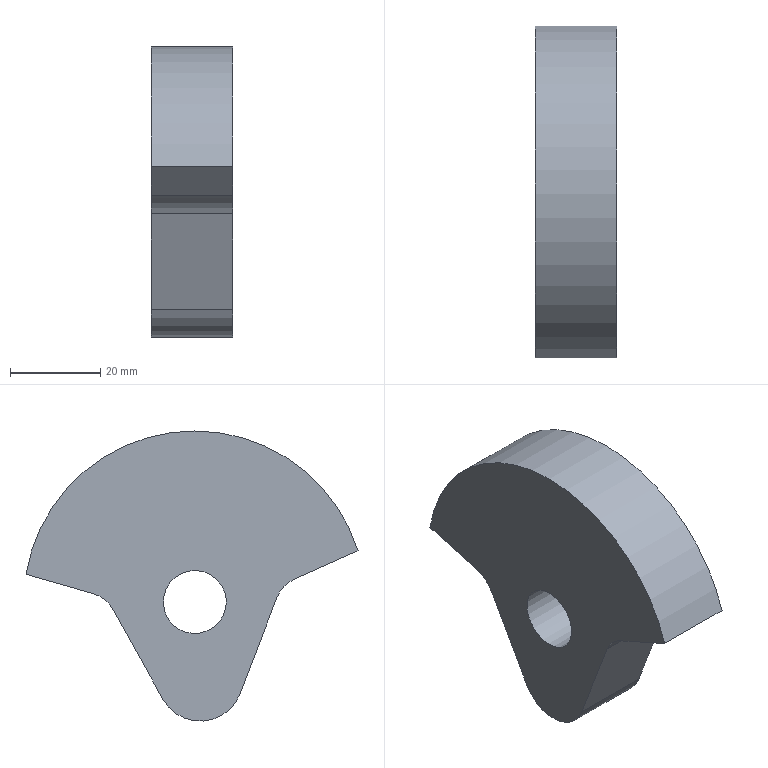Component | NX | TURNTABLE | 1 solid | 11 faces | box 18 x 73.75 x 64.46 mm | volume 45751 mm3 | plane 6 | cylinder 5 | commonest cylinder face diameters 14.905 x2 76 x1 19 x1 14 x1
STEP:
#1=CARTESIAN_POINT('',(0.,0.,0.));
#2=DIRECTION('',(0.,0.,1.));
#3=DIRECTION('',(1.,0.,0.));
#4=AXIS2_PLACEMENT_3D('',#1,#2,#3);
#5=CARTESIAN_POINT('',(-62.75,37.501,129.137));
#6=VERTEX_POINT('',#5);
#7=CARTESIAN_POINT('',(-62.75,-36.252,134.393));
#8=VERTEX_POINT('',#7);
#9=CARTESIAN_POINT('',(-62.75,0.,123.));
#10=DIRECTION('',(1.,0.,0.));
#11=DIRECTION('',(0.,0.9975,-0.07108));
#12=AXIS2_PLACEMENT_3D('',#9,#10,#11);
#13=CIRCLE('',#12,38.);
#14=CARTESIAN_POINT('',(-80.75,0.,123.));
#15=DIRECTION('',(1.,0.,0.));
#16=DIRECTION('',(0.,-0.07108,-0.9975));
#17=AXIS2_PLACEMENT_3D('',#14,#15,#16);
#18=CYLINDRICAL_SURFACE('',#17,38.);
#19=CARTESIAN_POINT('',(1.571,18.));
#20=DIRECTION('',(1.,0.));
#21=VECTOR('',#20,1.);
#22=LINE('',#19,#21);
#23=(GEOMETRIC_REPRESENTATION_CONTEXT(2)PARAMETRIC_REPRESENTATION_CONTEXT()REPRESENTATION_CONTEXT('',''));
#24=DEFINITIONAL_REPRESENTATION('',(#22),#23);
#25=PCURVE('',#18,#24);
#26=CARTESIAN_POINT('',(-62.75,0.,123.));
#27=DIRECTION('',(1.,0.,0.));
#28=DIRECTION('',(0.,-0.07108,-0.9975));
#29=AXIS2_PLACEMENT_3D('',#26,#27,#28);
#30=PLANE('',#29);
#31=CARTESIAN_POINT('',(0.,0.));
#32=DIRECTION('',(0.,1.));
#33=AXIS2_PLACEMENT_2D('',#31,#32);
#34=CIRCLE('',#33,38.);
#35=(GEOMETRIC_REPRESENTATION_CONTEXT(2)PARAMETRIC_REPRESENTATION_CONTEXT()REPRESENTATION_CONTEXT('',''));
#36=DEFINITIONAL_REPRESENTATION('',(#34),#35);
#37=PCURVE('',#30,#36);
#38=SURFACE_CURVE('',#13,(#25,#37),.PCURVE_S1.);
#39=EDGE_CURVE('',#6,#8,#38,.T.);
#40=ORIENTED_EDGE('',*,*,#39,.F.);
#41=CARTESIAN_POINT('',(-80.75,37.501,129.137));
#42=VERTEX_POINT('',#41);
#43=CARTESIAN_POINT('',(-80.75,37.501,129.137));
#44=DIRECTION('',(1.,0.,0.));
#45=VECTOR('',#44,1.);
#46=LINE('',#43,#45);
#47=CARTESIAN_POINT('',(1.804,0.));
#48=DIRECTION('',(0.,1.));
#49=VECTOR('',#48,1.);
#50=LINE('',#47,#49);
#51=(GEOMETRIC_REPRESENTATION_CONTEXT(2)PARAMETRIC_REPRESENTATION_CONTEXT()REPRESENTATION_CONTEXT('',''));
#52=DEFINITIONAL_REPRESENTATION('',(#50),#51);
#53=PCURVE('',#18,#52);
#54=CARTESIAN_POINT('',(-80.75,22.643,124.898));
#55=DIRECTION('',(0.,0.2744,-0.9616));
#56=DIRECTION('',(0.,-0.9616,-0.2744));
#57=AXIS2_PLACEMENT_3D('',#54,#55,#56);
#58=PLANE('',#57);
#59=CARTESIAN_POINT('',(-15.451,0.));
#60=DIRECTION('',(0.,-1.));
#61=VECTOR('',#60,1.);
#62=LINE('',#59,#61);
#63=(GEOMETRIC_REPRESENTATION_CONTEXT(2)PARAMETRIC_REPRESENTATION_CONTEXT()REPRESENTATION_CONTEXT('',''));
#64=DEFINITIONAL_REPRESENTATION('',(#62),#63);
#65=PCURVE('',#58,#64);
#66=SURFACE_CURVE('',#46,(#53,#65),.PCURVE_S1.);
#67=EDGE_CURVE('',#42,#6,#66,.T.);
#68=ORIENTED_EDGE('',*,*,#67,.F.);
#69=CARTESIAN_POINT('',(-80.75,-36.252,134.393));
#70=VERTEX_POINT('',#69);
#71=CARTESIAN_POINT('',(-80.75,0.,123.));
#72=DIRECTION('',(1.,0.,0.));
#73=DIRECTION('',(0.,0.9975,-0.07108));
#74=AXIS2_PLACEMENT_3D('',#71,#72,#73);
#75=CIRCLE('',#74,38.);
#76=CARTESIAN_POINT('',(1.571,0.));
#77=DIRECTION('',(1.,0.));
#78=VECTOR('',#77,1.);
#79=LINE('',#76,#78);
#80=(GEOMETRIC_REPRESENTATION_CONTEXT(2)PARAMETRIC_REPRESENTATION_CONTEXT()REPRESENTATION_CONTEXT('',''));
#81=DEFINITIONAL_REPRESENTATION('',(#79),#80);
#82=PCURVE('',#18,#81);
#83=CARTESIAN_POINT('',(-80.75,0.,123.));
#84=DIRECTION('',(1.,0.,0.));
#85=DIRECTION('',(0.,-0.07108,-0.9975));
#86=AXIS2_PLACEMENT_3D('',#83,#84,#85);
#87=PLANE('',#86);
#88=CARTESIAN_POINT('',(0.,0.));
#89=DIRECTION('',(0.,1.));
#90=AXIS2_PLACEMENT_2D('',#88,#89);
#91=CIRCLE('',#90,38.);
#92=(GEOMETRIC_REPRESENTATION_CONTEXT(2)PARAMETRIC_REPRESENTATION_CONTEXT()REPRESENTATION_CONTEXT('',''));
#93=DEFINITIONAL_REPRESENTATION('',(#91),#92);
#94=PCURVE('',#87,#93);
#95=SURFACE_CURVE('',#75,(#82,#94),.PCURVE_S1.);
#96=EDGE_CURVE('',#42,#70,#95,.T.);
#97=ORIENTED_EDGE('',*,*,#96,.T.);
#98=CARTESIAN_POINT('',(-80.75,-36.252,134.393));
#99=DIRECTION('',(1.,0.,0.));
#100=VECTOR('',#99,1.);
#101=LINE('',#98,#100);
#102=CARTESIAN_POINT('',(4.479,0.));
#103=DIRECTION('',(0.,1.));
#104=VECTOR('',#103,1.);
#105=LINE('',#102,#104);
#106=(GEOMETRIC_REPRESENTATION_CONTEXT(2)PARAMETRIC_REPRESENTATION_CONTEXT()REPRESENTATION_CONTEXT('',''));
#107=DEFINITIONAL_REPRESENTATION('',(#105),#106);
#108=PCURVE('',#18,#107);
#109=CARTESIAN_POINT('',(-80.75,-36.252,134.393));
#110=DIRECTION('',(0.,-0.4079,-0.913));
#111=DIRECTION('',(0.,-0.913,0.4079));
#112=AXIS2_PLACEMENT_3D('',#109,#110,#111);
#113=PLANE('',#112);
#114=CARTESIAN_POINT('',(0.,0.));
#115=DIRECTION('',(0.,-1.));
#116=VECTOR('',#115,1.);
#117=LINE('',#114,#116);
#118=(GEOMETRIC_REPRESENTATION_CONTEXT(2)PARAMETRIC_REPRESENTATION_CONTEXT()REPRESENTATION_CONTEXT('',''));
#119=DEFINITIONAL_REPRESENTATION('',(#117),#118);
#120=PCURVE('',#113,#119);
#121=SURFACE_CURVE('',#101,(#108,#120),.PCURVE_S1.);
#122=EDGE_CURVE('',#70,#8,#121,.T.);
#123=ORIENTED_EDGE('',*,*,#122,.T.);
#124=EDGE_LOOP('',(#40,#68,#97,#123));
#125=FACE_BOUND('',#124,.T.);
#126=ADVANCED_FACE('',(#125),#18,.T.);
#127=CARTESIAN_POINT('',(-62.75,-22.145,128.09));
#128=VERTEX_POINT('',#127);
#129=CARTESIAN_POINT('',(-62.75,-36.252,134.393));
#130=DIRECTION('',(0.,0.913,-0.4079));
#131=VECTOR('',#130,1.);
#132=LINE('',#129,#131);
#133=CARTESIAN_POINT('',(0.,-18.));
#134=DIRECTION('',(-1.,0.));
#135=VECTOR('',#134,1.);
#136=LINE('',#133,#135);
#137=(GEOMETRIC_REPRESENTATION_CONTEXT(2)PARAMETRIC_REPRESENTATION_CONTEXT()REPRESENTATION_CONTEXT('',''));
#138=DEFINITIONAL_REPRESENTATION('',(#136),#137);
#139=PCURVE('',#113,#138);
#140=CARTESIAN_POINT('',(-8.787,-36.97));
#141=DIRECTION('',(0.342,0.9397));
#142=VECTOR('',#141,1.);
#143=LINE('',#140,#142);
#144=(GEOMETRIC_REPRESENTATION_CONTEXT(2)PARAMETRIC_REPRESENTATION_CONTEXT()REPRESENTATION_CONTEXT('',''));
#145=DEFINITIONAL_REPRESENTATION('',(#143),#144);
#146=PCURVE('',#30,#145);
#147=SURFACE_CURVE('',#132,(#139,#146),.PCURVE_S1.);
#148=EDGE_CURVE('',#8,#128,#147,.T.);
#149=ORIENTED_EDGE('',*,*,#148,.F.);
#150=ORIENTED_EDGE('',*,*,#122,.F.);
#151=CARTESIAN_POINT('',(-80.75,-22.145,128.09));
#152=VERTEX_POINT('',#151);
#153=CARTESIAN_POINT('',(-80.75,-36.252,134.393));
#154=DIRECTION('',(0.,0.913,-0.4079));
#155=VECTOR('',#154,1.);
#156=LINE('',#153,#155);
#157=CARTESIAN_POINT('',(0.,0.));
#158=DIRECTION('',(-1.,0.));
#159=VECTOR('',#158,1.);
#160=LINE('',#157,#159);
#161=(GEOMETRIC_REPRESENTATION_CONTEXT(2)PARAMETRIC_REPRESENTATION_CONTEXT()REPRESENTATION_CONTEXT('',''));
#162=DEFINITIONAL_REPRESENTATION('',(#160),#161);
#163=PCURVE('',#113,#162);
#164=CARTESIAN_POINT('',(-8.787,-36.97));
#165=DIRECTION('',(0.342,0.9397));
#166=VECTOR('',#165,1.);
#167=LINE('',#164,#166);
#168=(GEOMETRIC_REPRESENTATION_CONTEXT(2)PARAMETRIC_REPRESENTATION_CONTEXT()REPRESENTATION_CONTEXT('',''));
#169=DEFINITIONAL_REPRESENTATION('',(#167),#168);
#170=PCURVE('',#87,#169);
#171=SURFACE_CURVE('',#156,(#163,#170),.PCURVE_S1.);
#172=EDGE_CURVE('',#70,#152,#171,.T.);
#173=ORIENTED_EDGE('',*,*,#172,.T.);
#174=CARTESIAN_POINT('',(-80.75,-22.145,128.09));
#175=DIRECTION('',(1.,0.,0.));
#176=VECTOR('',#175,1.);
#177=LINE('',#174,#176);
#178=CARTESIAN_POINT('',(-15.451,0.));
#179=DIRECTION('',(0.,-1.));
#180=VECTOR('',#179,1.);
#181=LINE('',#178,#180);
#182=(GEOMETRIC_REPRESENTATION_CONTEXT(2)PARAMETRIC_REPRESENTATION_CONTEXT()REPRESENTATION_CONTEXT('',''));
#183=DEFINITIONAL_REPRESENTATION('',(#181),#182);
#184=PCURVE('',#113,#183);
#185=CARTESIAN_POINT('',(-80.75,-25.186,121.286));
#186=DIRECTION('',(1.,0.,0.));
#187=DIRECTION('',(0.,-0.07108,-0.9975));
#188=AXIS2_PLACEMENT_3D('',#185,#186,#187);
#189=CYLINDRICAL_SURFACE('',#188,7.452);
#190=CARTESIAN_POINT('',(2.793,0.));
#191=DIRECTION('',(0.,1.));
#192=VECTOR('',#191,1.);
#193=LINE('',#190,#192);
#194=(GEOMETRIC_REPRESENTATION_CONTEXT(2)PARAMETRIC_REPRESENTATION_CONTEXT()REPRESENTATION_CONTEXT('',''));
#195=DEFINITIONAL_REPRESENTATION('',(#193),#194);
#196=PCURVE('',#189,#195);
#197=SURFACE_CURVE('',#177,(#184,#196),.PCURVE_S1.);
#198=EDGE_CURVE('',#152,#128,#197,.T.);
#199=ORIENTED_EDGE('',*,*,#198,.T.);
#200=EDGE_LOOP('',(#149,#150,#173,#199));
#201=FACE_BOUND('',#200,.T.);
#202=ADVANCED_FACE('',(#201),#113,.T.);
#203=CARTESIAN_POINT('',(-80.75,-18.225,123.947));
#204=VERTEX_POINT('',#203);
#205=CARTESIAN_POINT('',(-62.75,-18.225,123.947));
#206=VERTEX_POINT('',#205);
#207=CARTESIAN_POINT('',(-80.75,-18.225,123.947));
#208=DIRECTION('',(1.,0.,0.));
#209=VECTOR('',#208,1.);
#210=LINE('',#207,#209);
#211=CARTESIAN_POINT('',(2.007,0.));
#212=DIRECTION('',(0.,1.));
#213=VECTOR('',#212,1.);
#214=LINE('',#211,#213);
#215=(GEOMETRIC_REPRESENTATION_CONTEXT(2)PARAMETRIC_REPRESENTATION_CONTEXT()REPRESENTATION_CONTEXT('',''));
#216=DEFINITIONAL_REPRESENTATION('',(#214),#215);
#217=PCURVE('',#189,#216);
#218=CARTESIAN_POINT('',(-80.75,-18.225,123.947));
#219=DIRECTION('',(0.,-0.9341,-0.3571));
#220=DIRECTION('',(0.,-0.3571,0.9341));
#221=AXIS2_PLACEMENT_3D('',#218,#219,#220);
#222=PLANE('',#221);
#223=CARTESIAN_POINT('',(0.,0.));
#224=DIRECTION('',(0.,-1.));
#225=VECTOR('',#224,1.);
#226=LINE('',#223,#225);
#227=(GEOMETRIC_REPRESENTATION_CONTEXT(2)PARAMETRIC_REPRESENTATION_CONTEXT()REPRESENTATION_CONTEXT('',''));
#228=DEFINITIONAL_REPRESENTATION('',(#226),#227);
#229=PCURVE('',#222,#228);
#230=SURFACE_CURVE('',#210,(#217,#229),.PCURVE_S1.);
#231=EDGE_CURVE('',#204,#206,#230,.T.);
#232=ORIENTED_EDGE('',*,*,#231,.F.);
#233=CARTESIAN_POINT('',(-80.75,-25.186,121.286));
#234=DIRECTION('',(-1.,0.,0.));
#235=DIRECTION('',(0.,0.9975,-0.07108));
#236=AXIS2_PLACEMENT_3D('',#233,#234,#235);
#237=CIRCLE('',#236,7.452);
#238=CARTESIAN_POINT('',(7.854,0.));
#239=DIRECTION('',(-1.,0.));
#240=VECTOR('',#239,1.);
#241=LINE('',#238,#240);
#242=(GEOMETRIC_REPRESENTATION_CONTEXT(2)PARAMETRIC_REPRESENTATION_CONTEXT()REPRESENTATION_CONTEXT('',''));
#243=DEFINITIONAL_REPRESENTATION('',(#241),#242);
#244=PCURVE('',#189,#243);
#245=CARTESIAN_POINT('',(3.5,-17.548));
#246=CARTESIAN_POINT('',(16.408,-17.548));
#247=CARTESIAN_POINT('',(9.954,-28.726));
#248=CARTESIAN_POINT('',(3.5,-39.905));
#249=CARTESIAN_POINT('',(-2.954,-28.726));
#250=CARTESIAN_POINT('',(-9.408,-17.548));
#251=CARTESIAN_POINT('',(3.5,-17.548));
#252=(BOUNDED_CURVE()B_SPLINE_CURVE(2,(#245,#246,#247,#248,#249,#250,#251),.UNSPECIFIED.,.T.,.F.)B_SPLINE_CURVE_WITH_KNOTS((1,2,2,2,2,1),(-2.094,0.,2.094,4.189,6.283,8.378),.UNSPECIFIED.)CURVE()GEOMETRIC_REPRESENTATION_ITEM()RATIONAL_B_SPLINE_CURVE((1.,0.5,1.,0.5,1.,0.5,1.))REPRESENTATION_ITEM(''));
#253=(GEOMETRIC_REPRESENTATION_CONTEXT(2)PARAMETRIC_REPRESENTATION_CONTEXT()REPRESENTATION_CONTEXT('',''));
#254=DEFINITIONAL_REPRESENTATION('',(#252),#253);
#255=PCURVE('',#87,#254);
#256=SURFACE_CURVE('',#237,(#244,#255),.PCURVE_S1.);
#257=EDGE_CURVE('',#152,#204,#256,.T.);
#258=ORIENTED_EDGE('',*,*,#257,.F.);
#259=ORIENTED_EDGE('',*,*,#198,.T.);
#260=CARTESIAN_POINT('',(-62.75,-25.186,121.286));
#261=DIRECTION('',(-1.,0.,0.));
#262=DIRECTION('',(0.,0.9975,-0.07108));
#263=AXIS2_PLACEMENT_3D('',#260,#261,#262);
#264=CIRCLE('',#263,7.452);
#265=CARTESIAN_POINT('',(7.854,18.));
#266=DIRECTION('',(-1.,0.));
#267=VECTOR('',#266,1.);
#268=LINE('',#265,#267);
#269=(GEOMETRIC_REPRESENTATION_CONTEXT(2)PARAMETRIC_REPRESENTATION_CONTEXT()REPRESENTATION_CONTEXT('',''));
#270=DEFINITIONAL_REPRESENTATION('',(#268),#269);
#271=PCURVE('',#189,#270);
#272=CARTESIAN_POINT('',(3.5,-17.548));
#273=CARTESIAN_POINT('',(16.408,-17.548));
#274=CARTESIAN_POINT('',(9.954,-28.726));
#275=CARTESIAN_POINT('',(3.5,-39.905));
#276=CARTESIAN_POINT('',(-2.954,-28.726));
#277=CARTESIAN_POINT('',(-9.408,-17.548));
#278=CARTESIAN_POINT('',(3.5,-17.548));
#279=(BOUNDED_CURVE()B_SPLINE_CURVE(2,(#272,#273,#274,#275,#276,#277,#278),.UNSPECIFIED.,.T.,.F.)B_SPLINE_CURVE_WITH_KNOTS((1,2,2,2,2,1),(-2.094,0.,2.094,4.189,6.283,8.378),.UNSPECIFIED.)CURVE()GEOMETRIC_REPRESENTATION_ITEM()RATIONAL_B_SPLINE_CURVE((1.,0.5,1.,0.5,1.,0.5,1.))REPRESENTATION_ITEM(''));
#280=(GEOMETRIC_REPRESENTATION_CONTEXT(2)PARAMETRIC_REPRESENTATION_CONTEXT()REPRESENTATION_CONTEXT('',''));
#281=DEFINITIONAL_REPRESENTATION('',(#279),#280);
#282=PCURVE('',#30,#281);
#283=SURFACE_CURVE('',#264,(#271,#282),.PCURVE_S1.);
#284=EDGE_CURVE('',#128,#206,#283,.T.);
#285=ORIENTED_EDGE('',*,*,#284,.T.);
#286=EDGE_LOOP('',(#232,#258,#259,#285));
#287=FACE_BOUND('',#286,.F.);
#288=ADVANCED_FACE('',(#287),#189,.F.);
#289=CARTESIAN_POINT('',(-62.75,-10.082,102.65));
#290=VERTEX_POINT('',#289);
#291=CARTESIAN_POINT('',(-62.75,-18.225,123.947));
#292=DIRECTION('',(0.,0.3571,-0.9341));
#293=VECTOR('',#292,1.);
#294=LINE('',#291,#293);
#295=CARTESIAN_POINT('',(0.,-18.));
#296=DIRECTION('',(-1.,0.));
#297=VECTOR('',#296,1.);
#298=LINE('',#295,#297);
#299=(GEOMETRIC_REPRESENTATION_CONTEXT(2)PARAMETRIC_REPRESENTATION_CONTEXT()REPRESENTATION_CONTEXT('',''));
#300=DEFINITIONAL_REPRESENTATION('',(#298),#299);
#301=PCURVE('',#222,#300);
#302=CARTESIAN_POINT('',(0.3505,-18.246));
#303=DIRECTION('',(0.9063,0.4226));
#304=VECTOR('',#303,1.);
#305=LINE('',#302,#304);
#306=(GEOMETRIC_REPRESENTATION_CONTEXT(2)PARAMETRIC_REPRESENTATION_CONTEXT()REPRESENTATION_CONTEXT('',''));
#307=DEFINITIONAL_REPRESENTATION('',(#305),#306);
#308=PCURVE('',#30,#307);
#309=SURFACE_CURVE('',#294,(#301,#308),.PCURVE_S1.);
#310=EDGE_CURVE('',#206,#290,#309,.T.);
#311=ORIENTED_EDGE('',*,*,#310,.F.);
#312=ORIENTED_EDGE('',*,*,#231,.F.);
#313=CARTESIAN_POINT('',(-80.75,-10.082,102.65));
#314=VERTEX_POINT('',#313);
#315=CARTESIAN_POINT('',(-80.75,-18.225,123.947));
#316=DIRECTION('',(0.,0.3571,-0.9341));
#317=VECTOR('',#316,1.);
#318=LINE('',#315,#317);
#319=CARTESIAN_POINT('',(0.,0.));
#320=DIRECTION('',(-1.,0.));
#321=VECTOR('',#320,1.);
#322=LINE('',#319,#321);
#323=(GEOMETRIC_REPRESENTATION_CONTEXT(2)PARAMETRIC_REPRESENTATION_CONTEXT()REPRESENTATION_CONTEXT('',''));
#324=DEFINITIONAL_REPRESENTATION('',(#322),#323);
#325=PCURVE('',#222,#324);
#326=CARTESIAN_POINT('',(0.3505,-18.246));
#327=DIRECTION('',(0.9063,0.4226));
#328=VECTOR('',#327,1.);
#329=LINE('',#326,#328);
#330=(GEOMETRIC_REPRESENTATION_CONTEXT(2)PARAMETRIC_REPRESENTATION_CONTEXT()REPRESENTATION_CONTEXT('',''));
#331=DEFINITIONAL_REPRESENTATION('',(#329),#330);
#332=PCURVE('',#87,#331);
#333=SURFACE_CURVE('',#318,(#325,#332),.PCURVE_S1.);
#334=EDGE_CURVE('',#204,#314,#333,.T.);
#335=ORIENTED_EDGE('',*,*,#334,.T.);
#336=CARTESIAN_POINT('',(-80.75,-10.082,102.65));
#337=DIRECTION('',(1.,0.,0.));
#338=VECTOR('',#337,1.);
#339=LINE('',#336,#338);
#340=CARTESIAN_POINT('',(-22.801,0.));
#341=DIRECTION('',(0.,-1.));
#342=VECTOR('',#341,1.);
#343=LINE('',#340,#342);
#344=(GEOMETRIC_REPRESENTATION_CONTEXT(2)PARAMETRIC_REPRESENTATION_CONTEXT()REPRESENTATION_CONTEXT('',''));
#345=DEFINITIONAL_REPRESENTATION('',(#343),#344);
#346=PCURVE('',#222,#345);
#347=CARTESIAN_POINT('',(-80.75,-1.208,106.043));
#348=DIRECTION('',(1.,0.,0.));
#349=DIRECTION('',(0.,-0.07108,-0.9975));
#350=AXIS2_PLACEMENT_3D('',#347,#348,#349);
#351=CYLINDRICAL_SURFACE('',#350,9.5);
#352=CARTESIAN_POINT('',(-1.134,0.));
#353=DIRECTION('',(0.,1.));
#354=VECTOR('',#353,1.);
#355=LINE('',#352,#354);
#356=(GEOMETRIC_REPRESENTATION_CONTEXT(2)PARAMETRIC_REPRESENTATION_CONTEXT()REPRESENTATION_CONTEXT('',''));
#357=DEFINITIONAL_REPRESENTATION('',(#355),#356);
#358=PCURVE('',#351,#357);
#359=SURFACE_CURVE('',#339,(#346,#358),.PCURVE_S1.);
#360=EDGE_CURVE('',#314,#290,#359,.T.);
#361=ORIENTED_EDGE('',*,*,#360,.T.);
#362=EDGE_LOOP('',(#311,#312,#335,#361));
#363=FACE_BOUND('',#362,.T.);
#364=ADVANCED_FACE('',(#363),#222,.T.);
#365=CARTESIAN_POINT('',(-62.75,7.094,101.426));
#366=VERTEX_POINT('',#365);
#367=CARTESIAN_POINT('',(-62.75,-1.208,106.043));
#368=DIRECTION('',(1.,0.,0.));
#369=DIRECTION('',(0.,0.9975,-0.07108));
#370=AXIS2_PLACEMENT_3D('',#367,#368,#369);
#371=CIRCLE('',#370,9.5);
#372=CARTESIAN_POINT('',(-4.712,18.));
#373=DIRECTION('',(1.,0.));
#374=VECTOR('',#373,1.);
#375=LINE('',#372,#374);
#376=(GEOMETRIC_REPRESENTATION_CONTEXT(2)PARAMETRIC_REPRESENTATION_CONTEXT()REPRESENTATION_CONTEXT('',''));
#377=DEFINITIONAL_REPRESENTATION('',(#375),#376);
#378=PCURVE('',#351,#377);
#379=CARTESIAN_POINT('',(17.,-0.));
#380=DIRECTION('',(-0.,1.));
#381=AXIS2_PLACEMENT_2D('',#379,#380);
#382=CIRCLE('',#381,9.5);
#383=(GEOMETRIC_REPRESENTATION_CONTEXT(2)PARAMETRIC_REPRESENTATION_CONTEXT()REPRESENTATION_CONTEXT('',''));
#384=DEFINITIONAL_REPRESENTATION('',(#382),#383);
#385=PCURVE('',#30,#384);
#386=SURFACE_CURVE('',#371,(#378,#385),.PCURVE_S1.);
#387=EDGE_CURVE('',#290,#366,#386,.T.);
#388=ORIENTED_EDGE('',*,*,#387,.F.);
#389=ORIENTED_EDGE('',*,*,#360,.F.);
#390=CARTESIAN_POINT('',(-80.75,7.094,101.426));
#391=VERTEX_POINT('',#390);
#392=CARTESIAN_POINT('',(-80.75,-1.208,106.043));
#393=DIRECTION('',(1.,0.,0.));
#394=DIRECTION('',(0.,0.9975,-0.07108));
#395=AXIS2_PLACEMENT_3D('',#392,#393,#394);
#396=CIRCLE('',#395,9.5);
#397=CARTESIAN_POINT('',(-4.712,0.));
#398=DIRECTION('',(1.,0.));
#399=VECTOR('',#398,1.);
#400=LINE('',#397,#399);
#401=(GEOMETRIC_REPRESENTATION_CONTEXT(2)PARAMETRIC_REPRESENTATION_CONTEXT()REPRESENTATION_CONTEXT('',''));
#402=DEFINITIONAL_REPRESENTATION('',(#400),#401);
#403=PCURVE('',#351,#402);
#404=CARTESIAN_POINT('',(17.,-0.));
#405=DIRECTION('',(-0.,1.));
#406=AXIS2_PLACEMENT_2D('',#404,#405);
#407=CIRCLE('',#406,9.5);
#408=(GEOMETRIC_REPRESENTATION_CONTEXT(2)PARAMETRIC_REPRESENTATION_CONTEXT()REPRESENTATION_CONTEXT('',''));
#409=DEFINITIONAL_REPRESENTATION('',(#407),#408);
#410=PCURVE('',#87,#409);
#411=SURFACE_CURVE('',#396,(#403,#410),.PCURVE_S1.);
#412=EDGE_CURVE('',#314,#391,#411,.T.);
#413=ORIENTED_EDGE('',*,*,#412,.T.);
#414=CARTESIAN_POINT('',(-80.75,7.094,101.426));
#415=DIRECTION('',(1.,0.,0.));
#416=VECTOR('',#415,1.);
#417=LINE('',#414,#416);
#418=CARTESIAN_POINT('',(1.134,0.));
#419=DIRECTION('',(0.,1.));
#420=VECTOR('',#419,1.);
#421=LINE('',#418,#420);
#422=(GEOMETRIC_REPRESENTATION_CONTEXT(2)PARAMETRIC_REPRESENTATION_CONTEXT()REPRESENTATION_CONTEXT('',''));
#423=DEFINITIONAL_REPRESENTATION('',(#421),#422);
#424=PCURVE('',#351,#423);
#425=CARTESIAN_POINT('',(-80.75,7.094,101.426));
#426=DIRECTION('',(0.,0.874,-0.486));
#427=DIRECTION('',(0.,-0.486,-0.874));
#428=AXIS2_PLACEMENT_3D('',#425,#426,#427);
#429=PLANE('',#428);
#430=CARTESIAN_POINT('',(-0.,0.));
#431=DIRECTION('',(0.,-1.));
#432=VECTOR('',#431,1.);
#433=LINE('',#430,#432);
#434=(GEOMETRIC_REPRESENTATION_CONTEXT(2)PARAMETRIC_REPRESENTATION_CONTEXT()REPRESENTATION_CONTEXT('',''));
#435=DEFINITIONAL_REPRESENTATION('',(#433),#434);
#436=PCURVE('',#429,#435);
#437=SURFACE_CURVE('',#417,(#424,#436),.PCURVE_S1.);
#438=EDGE_CURVE('',#391,#366,#437,.T.);
#439=ORIENTED_EDGE('',*,*,#438,.T.);
#440=EDGE_LOOP('',(#388,#389,#413,#439));
#441=FACE_BOUND('',#440,.T.);
#442=ADVANCED_FACE('',(#441),#351,.T.);
#443=CARTESIAN_POINT('',(-62.75,18.175,121.354));
#444=VERTEX_POINT('',#443);
#445=CARTESIAN_POINT('',(-62.75,7.094,101.426));
#446=DIRECTION('',(0.,0.486,0.874));
#447=VECTOR('',#446,1.);
#448=LINE('',#445,#447);
#449=CARTESIAN_POINT('',(0.,-18.));
#450=DIRECTION('',(-1.,0.));
#451=VECTOR('',#450,1.);
#452=LINE('',#449,#451);
#453=(GEOMETRIC_REPRESENTATION_CONTEXT(2)PARAMETRIC_REPRESENTATION_CONTEXT()REPRESENTATION_CONTEXT('',''));
#454=DEFINITIONAL_REPRESENTATION('',(#452),#453);
#455=PCURVE('',#429,#454);
#456=CARTESIAN_POINT('',(21.015,8.61));
#457=DIRECTION('',(-0.9063,0.4226));
#458=VECTOR('',#457,1.);
#459=LINE('',#456,#458);
#460=(GEOMETRIC_REPRESENTATION_CONTEXT(2)PARAMETRIC_REPRESENTATION_CONTEXT()REPRESENTATION_CONTEXT('',''));
#461=DEFINITIONAL_REPRESENTATION('',(#459),#460);
#462=PCURVE('',#30,#461);
#463=SURFACE_CURVE('',#448,(#455,#462),.PCURVE_S1.);
#464=EDGE_CURVE('',#366,#444,#463,.T.);
#465=ORIENTED_EDGE('',*,*,#464,.F.);
#466=ORIENTED_EDGE('',*,*,#438,.F.);
#467=CARTESIAN_POINT('',(-80.75,18.175,121.354));
#468=VERTEX_POINT('',#467);
#469=CARTESIAN_POINT('',(-80.75,7.094,101.426));
#470=DIRECTION('',(0.,0.486,0.874));
#471=VECTOR('',#470,1.);
#472=LINE('',#469,#471);
#473=CARTESIAN_POINT('',(0.,0.));
#474=DIRECTION('',(-1.,0.));
#475=VECTOR('',#474,1.);
#476=LINE('',#473,#475);
#477=(GEOMETRIC_REPRESENTATION_CONTEXT(2)PARAMETRIC_REPRESENTATION_CONTEXT()REPRESENTATION_CONTEXT('',''));
#478=DEFINITIONAL_REPRESENTATION('',(#476),#477);
#479=PCURVE('',#429,#478);
#480=CARTESIAN_POINT('',(21.015,8.61));
#481=DIRECTION('',(-0.9063,0.4226));
#482=VECTOR('',#481,1.);
#483=LINE('',#480,#482);
#484=(GEOMETRIC_REPRESENTATION_CONTEXT(2)PARAMETRIC_REPRESENTATION_CONTEXT()REPRESENTATION_CONTEXT('',''));
#485=DEFINITIONAL_REPRESENTATION('',(#483),#484);
#486=PCURVE('',#87,#485);
#487=SURFACE_CURVE('',#472,(#479,#486),.PCURVE_S1.);
#488=EDGE_CURVE('',#391,#468,#487,.T.);
#489=ORIENTED_EDGE('',*,*,#488,.T.);
#490=CARTESIAN_POINT('',(-80.75,18.175,121.354));
#491=DIRECTION('',(1.,0.,0.));
#492=VECTOR('',#491,1.);
#493=LINE('',#490,#492);
#494=CARTESIAN_POINT('',(-22.801,0.));
#495=DIRECTION('',(0.,-1.));
#496=VECTOR('',#495,1.);
#497=LINE('',#494,#496);
#498=(GEOMETRIC_REPRESENTATION_CONTEXT(2)PARAMETRIC_REPRESENTATION_CONTEXT()REPRESENTATION_CONTEXT('',''));
#499=DEFINITIONAL_REPRESENTATION('',(#497),#498);
#500=PCURVE('',#429,#499);
#501=CARTESIAN_POINT('',(-80.75,24.688,117.732));
#502=DIRECTION('',(1.,0.,0.));
#503=DIRECTION('',(0.,-0.07108,-0.9975));
#504=AXIS2_PLACEMENT_3D('',#501,#502,#503);
#505=CYLINDRICAL_SURFACE('',#504,7.452);
#506=CARTESIAN_POINT('',(4.276,0.));
#507=DIRECTION('',(0.,1.));
#508=VECTOR('',#507,1.);
#509=LINE('',#506,#508);
#510=(GEOMETRIC_REPRESENTATION_CONTEXT(2)PARAMETRIC_REPRESENTATION_CONTEXT()REPRESENTATION_CONTEXT('',''));
#511=DEFINITIONAL_REPRESENTATION('',(#509),#510);
#512=PCURVE('',#505,#511);
#513=SURFACE_CURVE('',#493,(#500,#512),.PCURVE_S1.);
#514=EDGE_CURVE('',#468,#444,#513,.T.);
#515=ORIENTED_EDGE('',*,*,#514,.T.);
#516=EDGE_LOOP('',(#465,#466,#489,#515));
#517=FACE_BOUND('',#516,.T.);
#518=ADVANCED_FACE('',(#517),#429,.T.);
#519=CARTESIAN_POINT('',(-80.75,22.643,124.898));
#520=VERTEX_POINT('',#519);
#521=CARTESIAN_POINT('',(-62.75,22.643,124.898));
#522=VERTEX_POINT('',#521);
#523=CARTESIAN_POINT('',(-80.75,22.643,124.898));
#524=DIRECTION('',(1.,0.,0.));
#525=VECTOR('',#524,1.);
#526=LINE('',#523,#525);
#527=CARTESIAN_POINT('',(3.491,0.));
#528=DIRECTION('',(0.,1.));
#529=VECTOR('',#528,1.);
#530=LINE('',#527,#529);
#531=(GEOMETRIC_REPRESENTATION_CONTEXT(2)PARAMETRIC_REPRESENTATION_CONTEXT()REPRESENTATION_CONTEXT('',''));
#532=DEFINITIONAL_REPRESENTATION('',(#530),#531);
#533=PCURVE('',#505,#532);
#534=CARTESIAN_POINT('',(0.,0.));
#535=DIRECTION('',(0.,-1.));
#536=VECTOR('',#535,1.);
#537=LINE('',#534,#536);
#538=(GEOMETRIC_REPRESENTATION_CONTEXT(2)PARAMETRIC_REPRESENTATION_CONTEXT()REPRESENTATION_CONTEXT('',''));
#539=DEFINITIONAL_REPRESENTATION('',(#537),#538);
#540=PCURVE('',#58,#539);
#541=SURFACE_CURVE('',#526,(#533,#540),.PCURVE_S1.);
#542=EDGE_CURVE('',#520,#522,#541,.T.);
#543=ORIENTED_EDGE('',*,*,#542,.F.);
#544=CARTESIAN_POINT('',(-80.75,24.688,117.732));
#545=DIRECTION('',(-1.,0.,0.));
#546=DIRECTION('',(0.,-0.9975,0.07108));
#547=AXIS2_PLACEMENT_3D('',#544,#545,#546);
#548=CIRCLE('',#547,7.452);
#549=CARTESIAN_POINT('',(4.712,0.));
#550=DIRECTION('',(-1.,0.));
#551=VECTOR('',#550,1.);
#552=LINE('',#549,#551);
#553=(GEOMETRIC_REPRESENTATION_CONTEXT(2)PARAMETRIC_REPRESENTATION_CONTEXT()REPRESENTATION_CONTEXT('',''));
#554=DEFINITIONAL_REPRESENTATION('',(#552),#553);
#555=PCURVE('',#505,#554);
#556=CARTESIAN_POINT('',(3.5,17.548));
#557=CARTESIAN_POINT('',(-9.408,17.548));
#558=CARTESIAN_POINT('',(-2.954,28.726));
#559=CARTESIAN_POINT('',(3.5,39.905));
#560=CARTESIAN_POINT('',(9.954,28.726));
#561=CARTESIAN_POINT('',(16.408,17.548));
#562=CARTESIAN_POINT('',(3.5,17.548));
#563=(BOUNDED_CURVE()B_SPLINE_CURVE(2,(#556,#557,#558,#559,#560,#561,#562),.UNSPECIFIED.,.T.,.F.)B_SPLINE_CURVE_WITH_KNOTS((1,2,2,2,2,1),(-2.094,0.,2.094,4.189,6.283,8.378),.UNSPECIFIED.)CURVE()GEOMETRIC_REPRESENTATION_ITEM()RATIONAL_B_SPLINE_CURVE((1.,0.5,1.,0.5,1.,0.5,1.))REPRESENTATION_ITEM(''));
#564=(GEOMETRIC_REPRESENTATION_CONTEXT(2)PARAMETRIC_REPRESENTATION_CONTEXT()REPRESENTATION_CONTEXT('',''));
#565=DEFINITIONAL_REPRESENTATION('',(#563),#564);
#566=PCURVE('',#87,#565);
#567=SURFACE_CURVE('',#548,(#555,#566),.PCURVE_S1.);
#568=EDGE_CURVE('',#468,#520,#567,.T.);
#569=ORIENTED_EDGE('',*,*,#568,.F.);
#570=ORIENTED_EDGE('',*,*,#514,.T.);
#571=CARTESIAN_POINT('',(-62.75,24.688,117.732));
#572=DIRECTION('',(-1.,0.,0.));
#573=DIRECTION('',(0.,-0.9975,0.07108));
#574=AXIS2_PLACEMENT_3D('',#571,#572,#573);
#575=CIRCLE('',#574,7.452);
#576=CARTESIAN_POINT('',(4.712,18.));
#577=DIRECTION('',(-1.,0.));
#578=VECTOR('',#577,1.);
#579=LINE('',#576,#578);
#580=(GEOMETRIC_REPRESENTATION_CONTEXT(2)PARAMETRIC_REPRESENTATION_CONTEXT()REPRESENTATION_CONTEXT('',''));
#581=DEFINITIONAL_REPRESENTATION('',(#579),#580);
#582=PCURVE('',#505,#581);
#583=CARTESIAN_POINT('',(3.5,17.548));
#584=CARTESIAN_POINT('',(-9.408,17.548));
#585=CARTESIAN_POINT('',(-2.954,28.726));
#586=CARTESIAN_POINT('',(3.5,39.905));
#587=CARTESIAN_POINT('',(9.954,28.726));
#588=CARTESIAN_POINT('',(16.408,17.548));
#589=CARTESIAN_POINT('',(3.5,17.548));
#590=(BOUNDED_CURVE()B_SPLINE_CURVE(2,(#583,#584,#585,#586,#587,#588,#589),.UNSPECIFIED.,.T.,.F.)B_SPLINE_CURVE_WITH_KNOTS((1,2,2,2,2,1),(-2.094,0.,2.094,4.189,6.283,8.378),.UNSPECIFIED.)CURVE()GEOMETRIC_REPRESENTATION_ITEM()RATIONAL_B_SPLINE_CURVE((1.,0.5,1.,0.5,1.,0.5,1.))REPRESENTATION_ITEM(''));
#591=(GEOMETRIC_REPRESENTATION_CONTEXT(2)PARAMETRIC_REPRESENTATION_CONTEXT()REPRESENTATION_CONTEXT('',''));
#592=DEFINITIONAL_REPRESENTATION('',(#590),#591);
#593=PCURVE('',#30,#592);
#594=SURFACE_CURVE('',#575,(#582,#593),.PCURVE_S1.);
#595=EDGE_CURVE('',#444,#522,#594,.T.);
#596=ORIENTED_EDGE('',*,*,#595,.T.);
#597=EDGE_LOOP('',(#543,#569,#570,#596));
#598=FACE_BOUND('',#597,.F.);
#599=ADVANCED_FACE('',(#598),#505,.F.);
#600=CARTESIAN_POINT('',(-62.75,22.643,124.898));
#601=DIRECTION('',(0.,0.9616,0.2744));
#602=VECTOR('',#601,1.);
#603=LINE('',#600,#602);
#604=CARTESIAN_POINT('',(0.,-18.));
#605=DIRECTION('',(-1.,0.));
#606=VECTOR('',#605,1.);
#607=LINE('',#604,#606);
#608=(GEOMETRIC_REPRESENTATION_CONTEXT(2)PARAMETRIC_REPRESENTATION_CONTEXT()REPRESENTATION_CONTEXT('',''));
#609=DEFINITIONAL_REPRESENTATION('',(#607),#608);
#610=PCURVE('',#58,#609);
#611=CARTESIAN_POINT('',(-3.503,22.451));
#612=DIRECTION('',(-0.342,0.9397));
#613=VECTOR('',#612,1.);
#614=LINE('',#611,#613);
#615=(GEOMETRIC_REPRESENTATION_CONTEXT(2)PARAMETRIC_REPRESENTATION_CONTEXT()REPRESENTATION_CONTEXT('',''));
#616=DEFINITIONAL_REPRESENTATION('',(#614),#615);
#617=PCURVE('',#30,#616);
#618=SURFACE_CURVE('',#603,(#610,#617),.PCURVE_S1.);
#619=EDGE_CURVE('',#522,#6,#618,.T.);
#620=ORIENTED_EDGE('',*,*,#619,.F.);
#621=ORIENTED_EDGE('',*,*,#542,.F.);
#622=CARTESIAN_POINT('',(-80.75,22.643,124.898));
#623=DIRECTION('',(0.,0.9616,0.2744));
#624=VECTOR('',#623,1.);
#625=LINE('',#622,#624);
#626=CARTESIAN_POINT('',(0.,0.));
#627=DIRECTION('',(-1.,0.));
#628=VECTOR('',#627,1.);
#629=LINE('',#626,#628);
#630=(GEOMETRIC_REPRESENTATION_CONTEXT(2)PARAMETRIC_REPRESENTATION_CONTEXT()REPRESENTATION_CONTEXT('',''));
#631=DEFINITIONAL_REPRESENTATION('',(#629),#630);
#632=PCURVE('',#58,#631);
#633=CARTESIAN_POINT('',(-3.503,22.451));
#634=DIRECTION('',(-0.342,0.9397));
#635=VECTOR('',#634,1.);
#636=LINE('',#633,#635);
#637=(GEOMETRIC_REPRESENTATION_CONTEXT(2)PARAMETRIC_REPRESENTATION_CONTEXT()REPRESENTATION_CONTEXT('',''));
#638=DEFINITIONAL_REPRESENTATION('',(#636),#637);
#639=PCURVE('',#87,#638);
#640=SURFACE_CURVE('',#625,(#632,#639),.PCURVE_S1.);
#641=EDGE_CURVE('',#520,#42,#640,.T.);
#642=ORIENTED_EDGE('',*,*,#641,.T.);
#643=ORIENTED_EDGE('',*,*,#67,.T.);
#644=EDGE_LOOP('',(#620,#621,#642,#643));
#645=FACE_BOUND('',#644,.T.);
#646=ADVANCED_FACE('',(#645),#58,.T.);
#647=CARTESIAN_POINT('',(-80.75,6.982,122.502));
#648=VERTEX_POINT('',#647);
#649=CARTESIAN_POINT('',(-80.75,0.,123.));
#650=DIRECTION('',(1.,0.,0.));
#651=DIRECTION('',(0.,0.9975,-0.07108));
#652=AXIS2_PLACEMENT_3D('',#649,#650,#651);
#653=CIRCLE('',#652,7.);
#654=CARTESIAN_POINT('',(-80.75,0.,123.));
#655=DIRECTION('',(1.,0.,0.));
#656=DIRECTION('',(0.,-0.07108,-0.9975));
#657=AXIS2_PLACEMENT_3D('',#654,#655,#656);
#658=CYLINDRICAL_SURFACE('',#657,7.);
#659=CARTESIAN_POINT('',(1.571,0.));
#660=DIRECTION('',(1.,0.));
#661=VECTOR('',#660,1.);
#662=LINE('',#659,#661);
#663=(GEOMETRIC_REPRESENTATION_CONTEXT(2)PARAMETRIC_REPRESENTATION_CONTEXT()REPRESENTATION_CONTEXT('',''));
#664=DEFINITIONAL_REPRESENTATION('',(#662),#663);
#665=PCURVE('',#658,#664);
#666=CARTESIAN_POINT('',(0.,0.));
#667=DIRECTION('',(0.,1.));
#668=AXIS2_PLACEMENT_2D('',#666,#667);
#669=CIRCLE('',#668,7.);
#670=(GEOMETRIC_REPRESENTATION_CONTEXT(2)PARAMETRIC_REPRESENTATION_CONTEXT()REPRESENTATION_CONTEXT('',''));
#671=DEFINITIONAL_REPRESENTATION('',(#669),#670);
#672=PCURVE('',#87,#671);
#673=SURFACE_CURVE('',#653,(#665,#672),.PCURVE_S1.);
#674=EDGE_CURVE('',#648,#648,#673,.T.);
#675=ORIENTED_EDGE('',*,*,#674,.T.);
#676=CARTESIAN_POINT('',(-62.75,6.982,122.502));
#677=VERTEX_POINT('',#676);
#678=CARTESIAN_POINT('',(-80.75,6.982,122.502));
#679=CARTESIAN_POINT('',(-62.75,6.982,122.502));
#680=B_SPLINE_CURVE_WITH_KNOTS('',1,(#678,#679),.UNSPECIFIED.,.F.,.F.,(2,2),(0.,18.),.PIECEWISE_BEZIER_KNOTS.);
#681=CARTESIAN_POINT('',(7.854,0.));
#682=DIRECTION('',(0.,1.));
#683=VECTOR('',#682,1.);
#684=LINE('',#681,#683);
#685=(GEOMETRIC_REPRESENTATION_CONTEXT(2)PARAMETRIC_REPRESENTATION_CONTEXT()REPRESENTATION_CONTEXT('',''));
#686=DEFINITIONAL_REPRESENTATION('',(#684),#685);
#687=PCURVE('',#658,#686);
#688=CARTESIAN_POINT('',(1.571,0.));
#689=DIRECTION('',(0.,1.));
#690=VECTOR('',#689,1.);
#691=LINE('',#688,#690);
#692=(GEOMETRIC_REPRESENTATION_CONTEXT(2)PARAMETRIC_REPRESENTATION_CONTEXT()REPRESENTATION_CONTEXT('',''));
#693=DEFINITIONAL_REPRESENTATION('',(#691),#692);
#694=PCURVE('',#658,#693);
#695=SEAM_CURVE('',#680,(#687,#694),.PCURVE_S1.);
#696=EDGE_CURVE('',#648,#677,#695,.T.);
#697=ORIENTED_EDGE('',*,*,#696,.T.);
#698=CARTESIAN_POINT('',(-62.75,0.,123.));
#699=DIRECTION('',(1.,0.,0.));
#700=DIRECTION('',(0.,0.9975,-0.07108));
#701=AXIS2_PLACEMENT_3D('',#698,#699,#700);
#702=CIRCLE('',#701,7.);
#703=CARTESIAN_POINT('',(1.571,18.));
#704=DIRECTION('',(1.,0.));
#705=VECTOR('',#704,1.);
#706=LINE('',#703,#705);
#707=(GEOMETRIC_REPRESENTATION_CONTEXT(2)PARAMETRIC_REPRESENTATION_CONTEXT()REPRESENTATION_CONTEXT('',''));
#708=DEFINITIONAL_REPRESENTATION('',(#706),#707);
#709=PCURVE('',#658,#708);
#710=CARTESIAN_POINT('',(0.,0.));
#711=DIRECTION('',(0.,1.));
#712=AXIS2_PLACEMENT_2D('',#710,#711);
#713=CIRCLE('',#712,7.);
#714=(GEOMETRIC_REPRESENTATION_CONTEXT(2)PARAMETRIC_REPRESENTATION_CONTEXT()REPRESENTATION_CONTEXT('',''));
#715=DEFINITIONAL_REPRESENTATION('',(#713),#714);
#716=PCURVE('',#30,#715);
#717=SURFACE_CURVE('',#702,(#709,#716),.PCURVE_S1.);
#718=EDGE_CURVE('',#677,#677,#717,.T.);
#719=ORIENTED_EDGE('',*,*,#718,.F.);
#720=ORIENTED_EDGE('',*,*,#696,.F.);
#721=EDGE_LOOP('',(#675,#697,#719,#720));
#722=FACE_BOUND('',#721,.F.);
#723=ADVANCED_FACE('',(#722),#658,.F.);
#724=ORIENTED_EDGE('',*,*,#96,.F.);
#725=ORIENTED_EDGE('',*,*,#641,.F.);
#726=ORIENTED_EDGE('',*,*,#568,.F.);
#727=ORIENTED_EDGE('',*,*,#488,.F.);
#728=ORIENTED_EDGE('',*,*,#412,.F.);
#729=ORIENTED_EDGE('',*,*,#334,.F.);
#730=ORIENTED_EDGE('',*,*,#257,.F.);
#731=ORIENTED_EDGE('',*,*,#172,.F.);
#732=EDGE_LOOP('',(#724,#725,#726,#727,#728,#729,#730,#731));
#733=FACE_BOUND('',#732,.T.);
#734=ORIENTED_EDGE('',*,*,#674,.T.);
#735=EDGE_LOOP('',(#734));
#736=FACE_BOUND('',#735,.T.);
#737=ADVANCED_FACE('',(#733,#736),#87,.F.);
#738=ORIENTED_EDGE('',*,*,#39,.T.);
#739=ORIENTED_EDGE('',*,*,#148,.T.);
#740=ORIENTED_EDGE('',*,*,#284,.T.);
#741=ORIENTED_EDGE('',*,*,#310,.T.);
#742=ORIENTED_EDGE('',*,*,#387,.T.);
#743=ORIENTED_EDGE('',*,*,#464,.T.);
#744=ORIENTED_EDGE('',*,*,#595,.T.);
#745=ORIENTED_EDGE('',*,*,#619,.T.);
#746=EDGE_LOOP('',(#738,#739,#740,#741,#742,#743,#744,#745));
#747=FACE_BOUND('',#746,.T.);
#748=ORIENTED_EDGE('',*,*,#718,.F.);
#749=EDGE_LOOP('',(#748));
#750=FACE_BOUND('',#749,.T.);
#751=ADVANCED_FACE('',(#747,#750),#30,.T.);
#752=CLOSED_SHELL('',(#126,#202,#288,#364,#442,#518,#599,#646,#723,#737,#751));
#753=MANIFOLD_SOLID_BREP('',#752);
#754=(LENGTH_UNIT()NAMED_UNIT(*)SI_UNIT(.MILLI.,.METRE.));
#755=UNCERTAINTY_MEASURE_WITH_UNIT(LENGTH_MEASURE(0.000001),#754,'','');
#756=(NAMED_UNIT(*)PLANE_ANGLE_UNIT()SI_UNIT($,.RADIAN.));
#757=(NAMED_UNIT(*)SI_UNIT($,.STERADIAN.)SOLID_ANGLE_UNIT());
#758=(GEOMETRIC_REPRESENTATION_CONTEXT(3)GLOBAL_UNCERTAINTY_ASSIGNED_CONTEXT((#755))GLOBAL_UNIT_ASSIGNED_CONTEXT((#754,#756,#757))REPRESENTATION_CONTEXT('',''));
#759=ADVANCED_BREP_SHAPE_REPRESENTATION('',(#4,#753),#758);